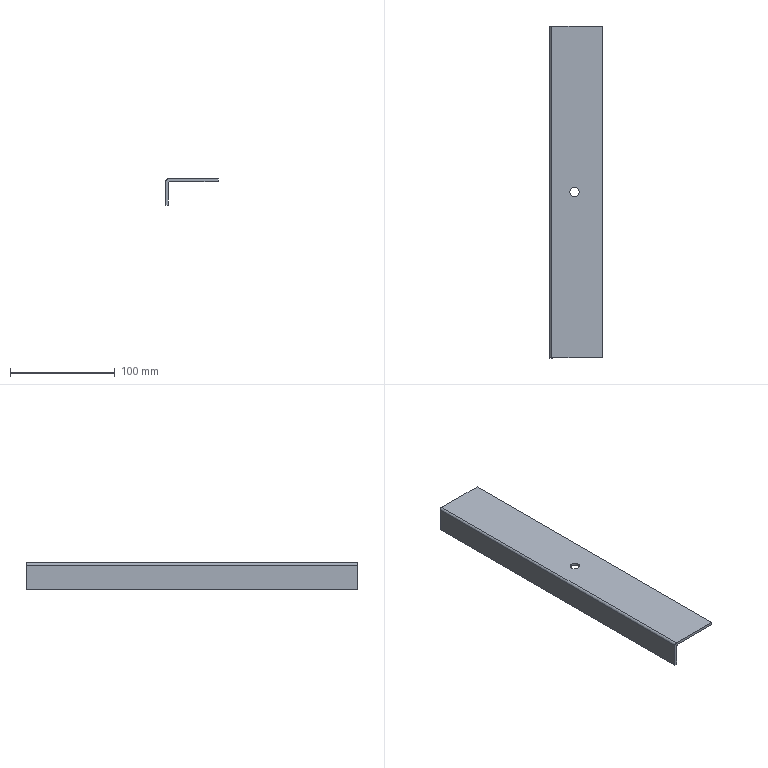Component | SolidWorks | FrameAssembly-1_FrameWeldment-1_SupportPlate-2 | 1 solid | 12 faces | box 50 x 317 x 25 mm | volume 57297 mm3 | plane 8 | cylinder 4 | commonest cylinder face diameters 9 x2 4 x2
STEP:
#1=CARTESIAN_POINT('',(-23.533,4.621,-1.339));
#2=VERTEX_POINT('',#1);
#3=CARTESIAN_POINT('',(-23.533,4.267,-1.339));
#4=VERTEX_POINT('',#3);
#5=CARTESIAN_POINT('',(-23.533,4.444,-1.339));
#6=DIRECTION('',(0.,0.,1.));
#7=DIRECTION('',(0.,-1.,0.));
#8=AXIS2_PLACEMENT_3D('',#5,#6,#7);
#9=CIRCLE('',#8,0.1772);
#10=EDGE_CURVE('',#2,#4,#9,.T.);
#11=ORIENTED_EDGE('',*,*,#10,.F.);
#12=CARTESIAN_POINT('',(-23.533,4.621,-1.24));
#13=VERTEX_POINT('',#12);
#14=CARTESIAN_POINT('',(-23.533,4.621,-1.24));
#15=DIRECTION('',(0.,0.,1.));
#16=VECTOR('',#15,39.37);
#17=LINE('',#14,#16);
#18=EDGE_CURVE('',#2,#13,#17,.T.);
#19=ORIENTED_EDGE('',*,*,#18,.T.);
#20=CARTESIAN_POINT('',(-23.533,4.267,-1.24));
#21=VERTEX_POINT('',#20);
#22=CARTESIAN_POINT('',(-23.533,4.444,-1.24));
#23=DIRECTION('',(0.,0.,1.));
#24=DIRECTION('',(0.,-1.,0.));
#25=AXIS2_PLACEMENT_3D('',#22,#23,#24);
#26=CIRCLE('',#25,0.1772);
#27=EDGE_CURVE('',#13,#21,#26,.T.);
#28=ORIENTED_EDGE('',*,*,#27,.T.);
#29=CARTESIAN_POINT('',(-23.533,4.267,-1.24));
#30=DIRECTION('',(0.,0.,1.));
#31=VECTOR('',#30,39.37);
#32=LINE('',#29,#31);
#33=EDGE_CURVE('',#4,#21,#32,.T.);
#34=ORIENTED_EDGE('',*,*,#33,.F.);
#35=EDGE_LOOP('',(#11,#19,#28,#34));
#36=FACE_OUTER_BOUND('',#35,.T.);
#37=CARTESIAN_POINT('',(-23.533,4.444,-1.24));
#38=DIRECTION('',(0.,0.,1.));
#39=DIRECTION('',(0.,-1.,0.));
#40=AXIS2_PLACEMENT_3D('',#37,#38,#39);
#41=CYLINDRICAL_SURFACE('',#40,0.1772);
#42=ADVANCED_FACE('',(#36),#41,.F.);
#43=CARTESIAN_POINT('',(-24.459,-1.796,-1.319));
#44=VERTEX_POINT('',#43);
#45=CARTESIAN_POINT('',(-24.459,-1.796,-2.224));
#46=VERTEX_POINT('',#45);
#47=CARTESIAN_POINT('',(-24.459,-1.796,-1.319));
#48=DIRECTION('',(-0.,-0.,-1.));
#49=VECTOR('',#48,39.37);
#50=LINE('',#47,#49);
#51=EDGE_CURVE('',#44,#46,#50,.T.);
#52=ORIENTED_EDGE('',*,*,#51,.F.);
#53=CARTESIAN_POINT('',(-24.459,10.684,-1.319));
#54=VERTEX_POINT('',#53);
#55=CARTESIAN_POINT('',(-24.459,10.684,-1.319));
#56=DIRECTION('',(0.,-1.,0.));
#57=VECTOR('',#56,39.37);
#58=LINE('',#55,#57);
#59=EDGE_CURVE('',#54,#44,#58,.T.);
#60=ORIENTED_EDGE('',*,*,#59,.F.);
#61=CARTESIAN_POINT('',(-24.459,10.684,-2.224));
#62=VERTEX_POINT('',#61);
#63=CARTESIAN_POINT('',(-24.459,10.684,-1.319));
#64=DIRECTION('',(-0.,-0.,-1.));
#65=VECTOR('',#64,39.37);
#66=LINE('',#63,#65);
#67=EDGE_CURVE('',#54,#62,#66,.T.);
#68=ORIENTED_EDGE('',*,*,#67,.T.);
#69=CARTESIAN_POINT('',(-24.459,10.684,-2.224));
#70=DIRECTION('',(0.,-1.,0.));
#71=VECTOR('',#70,39.37);
#72=LINE('',#69,#71);
#73=EDGE_CURVE('',#62,#46,#72,.T.);
#74=ORIENTED_EDGE('',*,*,#73,.T.);
#75=EDGE_LOOP('',(#52,#60,#68,#74));
#76=FACE_OUTER_BOUND('',#75,.T.);
#77=CARTESIAN_POINT('',(-24.459,10.684,-1.319));
#78=DIRECTION('',(-1.,-0.,0.));
#79=DIRECTION('',(0.,0.,1.));
#80=AXIS2_PLACEMENT_3D('',#77,#78,#79);
#81=PLANE('',#80);
#82=ADVANCED_FACE('',(#76),#81,.T.);
#83=CARTESIAN_POINT('',(-24.38,-1.796,-1.24));
#84=VERTEX_POINT('',#83);
#85=CARTESIAN_POINT('',(-24.38,-1.796,-1.319));
#86=DIRECTION('',(0.,-1.,0.));
#87=DIRECTION('',(0.,0.,-1.));
#88=AXIS2_PLACEMENT_3D('',#85,#86,#87);
#89=CIRCLE('',#88,0.07874);
#90=EDGE_CURVE('',#84,#44,#89,.T.);
#91=ORIENTED_EDGE('',*,*,#90,.F.);
#92=CARTESIAN_POINT('',(-24.38,10.684,-1.24));
#93=VERTEX_POINT('',#92);
#94=CARTESIAN_POINT('',(-24.38,10.684,-1.24));
#95=DIRECTION('',(0.,-1.,0.));
#96=VECTOR('',#95,39.37);
#97=LINE('',#94,#96);
#98=EDGE_CURVE('',#93,#84,#97,.T.);
#99=ORIENTED_EDGE('',*,*,#98,.F.);
#100=CARTESIAN_POINT('',(-24.38,10.684,-1.319));
#101=DIRECTION('',(0.,-1.,0.));
#102=DIRECTION('',(0.,0.,-1.));
#103=AXIS2_PLACEMENT_3D('',#100,#101,#102);
#104=CIRCLE('',#103,0.07874);
#105=EDGE_CURVE('',#93,#54,#104,.T.);
#106=ORIENTED_EDGE('',*,*,#105,.T.);
#107=ORIENTED_EDGE('',*,*,#59,.T.);
#108=EDGE_LOOP('',(#91,#99,#106,#107));
#109=FACE_OUTER_BOUND('',#108,.T.);
#110=CARTESIAN_POINT('',(-24.38,10.684,-1.319));
#111=DIRECTION('',(0.,-1.,0.));
#112=DIRECTION('',(0.,0.,-1.));
#113=AXIS2_PLACEMENT_3D('',#110,#111,#112);
#114=CYLINDRICAL_SURFACE('',#113,0.07874);
#115=ADVANCED_FACE('',(#109),#114,.T.);
#116=CARTESIAN_POINT('',(-23.533,4.444,-1.24));
#117=DIRECTION('',(0.,0.,1.));
#118=DIRECTION('',(0.,-1.,0.));
#119=AXIS2_PLACEMENT_3D('',#116,#117,#118);
#120=CIRCLE('',#119,0.1772);
#121=EDGE_CURVE('',#21,#13,#120,.T.);
#122=ORIENTED_EDGE('',*,*,#121,.F.);
#123=ORIENTED_EDGE('',*,*,#27,.F.);
#124=EDGE_LOOP('',(#122,#123));
#125=FACE_BOUND('',#124,.T.);
#126=CARTESIAN_POINT('',(-22.49,-1.796,-1.24));
#127=VERTEX_POINT('',#126);
#128=CARTESIAN_POINT('',(-22.49,-1.796,-1.24));
#129=DIRECTION('',(-1.,-0.,0.));
#130=VECTOR('',#129,39.37);
#131=LINE('',#128,#130);
#132=EDGE_CURVE('',#127,#84,#131,.T.);
#133=ORIENTED_EDGE('',*,*,#132,.F.);
#134=CARTESIAN_POINT('',(-22.49,10.684,-1.24));
#135=VERTEX_POINT('',#134);
#136=CARTESIAN_POINT('',(-22.49,10.684,-1.24));
#137=DIRECTION('',(0.,-1.,0.));
#138=VECTOR('',#137,39.37);
#139=LINE('',#136,#138);
#140=EDGE_CURVE('',#135,#127,#139,.T.);
#141=ORIENTED_EDGE('',*,*,#140,.F.);
#142=CARTESIAN_POINT('',(-22.49,10.684,-1.24));
#143=DIRECTION('',(-1.,-0.,0.));
#144=VECTOR('',#143,39.37);
#145=LINE('',#142,#144);
#146=EDGE_CURVE('',#135,#93,#145,.T.);
#147=ORIENTED_EDGE('',*,*,#146,.T.);
#148=ORIENTED_EDGE('',*,*,#98,.T.);
#149=EDGE_LOOP('',(#133,#141,#147,#148));
#150=FACE_OUTER_BOUND('',#149,.T.);
#151=CARTESIAN_POINT('',(-22.49,10.684,-1.24));
#152=DIRECTION('',(0.,0.,1.));
#153=DIRECTION('',(1.,0.,-0.));
#154=AXIS2_PLACEMENT_3D('',#151,#152,#153);
#155=PLANE('',#154);
#156=ADVANCED_FACE('',(#125,#150),#155,.T.);
#157=CARTESIAN_POINT('',(-22.49,-1.796,-1.339));
#158=VERTEX_POINT('',#157);
#159=CARTESIAN_POINT('',(-22.49,10.684,-1.339));
#160=VERTEX_POINT('',#159);
#161=CARTESIAN_POINT('',(-22.49,-1.796,-1.339));
#162=DIRECTION('',(-0.,1.,-0.));
#163=VECTOR('',#162,39.37);
#164=LINE('',#161,#163);
#165=EDGE_CURVE('',#158,#160,#164,.T.);
#166=ORIENTED_EDGE('',*,*,#165,.T.);
#167=CARTESIAN_POINT('',(-22.49,10.684,-2.224));
#168=DIRECTION('',(0.,0.,1.));
#169=VECTOR('',#168,39.37);
#170=LINE('',#167,#169);
#171=EDGE_CURVE('',#160,#135,#170,.T.);
#172=ORIENTED_EDGE('',*,*,#171,.T.);
#173=ORIENTED_EDGE('',*,*,#140,.T.);
#174=CARTESIAN_POINT('',(-22.49,-1.796,-2.224));
#175=DIRECTION('',(0.,0.,1.));
#176=VECTOR('',#175,39.37);
#177=LINE('',#174,#176);
#178=EDGE_CURVE('',#158,#127,#177,.T.);
#179=ORIENTED_EDGE('',*,*,#178,.F.);
#180=EDGE_LOOP('',(#166,#172,#173,#179));
#181=FACE_OUTER_BOUND('',#180,.T.);
#182=CARTESIAN_POINT('',(-22.49,10.684,-2.224));
#183=DIRECTION('',(1.,0.,-0.));
#184=DIRECTION('',(-0.,1.,-0.));
#185=AXIS2_PLACEMENT_3D('',#182,#183,#184);
#186=PLANE('',#185);
#187=ADVANCED_FACE('',(#181),#186,.T.);
#188=CARTESIAN_POINT('',(-24.36,-1.796,-2.224));
#189=VERTEX_POINT('',#188);
#190=CARTESIAN_POINT('',(-24.36,10.684,-2.224));
#191=VERTEX_POINT('',#190);
#192=CARTESIAN_POINT('',(-24.36,-1.796,-2.224));
#193=DIRECTION('',(-0.,1.,-0.));
#194=VECTOR('',#193,39.37);
#195=LINE('',#192,#194);
#196=EDGE_CURVE('',#189,#191,#195,.T.);
#197=ORIENTED_EDGE('',*,*,#196,.F.);
#198=CARTESIAN_POINT('',(-24.459,-1.796,-2.224));
#199=DIRECTION('',(1.,0.,-0.));
#200=VECTOR('',#199,39.37);
#201=LINE('',#198,#200);
#202=EDGE_CURVE('',#46,#189,#201,.T.);
#203=ORIENTED_EDGE('',*,*,#202,.F.);
#204=ORIENTED_EDGE('',*,*,#73,.F.);
#205=CARTESIAN_POINT('',(-24.459,10.684,-2.224));
#206=DIRECTION('',(1.,0.,-0.));
#207=VECTOR('',#206,39.37);
#208=LINE('',#205,#207);
#209=EDGE_CURVE('',#62,#191,#208,.T.);
#210=ORIENTED_EDGE('',*,*,#209,.T.);
#211=EDGE_LOOP('',(#197,#203,#204,#210));
#212=FACE_OUTER_BOUND('',#211,.T.);
#213=CARTESIAN_POINT('',(-24.459,10.684,-2.224));
#214=DIRECTION('',(-0.,-0.,-1.));
#215=DIRECTION('',(-0.,1.,-0.));
#216=AXIS2_PLACEMENT_3D('',#213,#214,#215);
#217=PLANE('',#216);
#218=ADVANCED_FACE('',(#212),#217,.T.);
#219=ORIENTED_EDGE('',*,*,#171,.F.);
#220=CARTESIAN_POINT('',(-24.281,10.684,-1.339));
#221=VERTEX_POINT('',#220);
#222=CARTESIAN_POINT('',(-24.281,10.684,-1.339));
#223=DIRECTION('',(1.,0.,-0.));
#224=VECTOR('',#223,39.37);
#225=LINE('',#222,#224);
#226=EDGE_CURVE('',#221,#160,#225,.T.);
#227=ORIENTED_EDGE('',*,*,#226,.F.);
#228=CARTESIAN_POINT('',(-24.36,10.684,-1.417));
#229=VERTEX_POINT('',#228);
#230=CARTESIAN_POINT('',(-24.281,10.684,-1.417));
#231=DIRECTION('',(-0.,1.,-0.));
#232=DIRECTION('',(0.,0.,1.));
#233=AXIS2_PLACEMENT_3D('',#230,#231,#232);
#234=CIRCLE('',#233,0.07874);
#235=EDGE_CURVE('',#229,#221,#234,.T.);
#236=ORIENTED_EDGE('',*,*,#235,.F.);
#237=CARTESIAN_POINT('',(-24.36,10.684,-2.224));
#238=DIRECTION('',(0.,0.,1.));
#239=VECTOR('',#238,39.37);
#240=LINE('',#237,#239);
#241=EDGE_CURVE('',#191,#229,#240,.T.);
#242=ORIENTED_EDGE('',*,*,#241,.F.);
#243=ORIENTED_EDGE('',*,*,#209,.F.);
#244=ORIENTED_EDGE('',*,*,#67,.F.);
#245=ORIENTED_EDGE('',*,*,#105,.F.);
#246=ORIENTED_EDGE('',*,*,#146,.F.);
#247=EDGE_LOOP('',(#219,#227,#236,#242,#243,#244,#245,#246));
#248=FACE_OUTER_BOUND('',#247,.T.);
#249=CARTESIAN_POINT('',(-24.38,10.684,-1.319));
#250=DIRECTION('',(0.,-1.,0.));
#251=DIRECTION('',(-0.,-0.,-1.));
#252=AXIS2_PLACEMENT_3D('',#249,#250,#251);
#253=PLANE('',#252);
#254=ADVANCED_FACE('',(#248),#253,.F.);
#255=CARTESIAN_POINT('',(-24.281,-1.796,-1.339));
#256=VERTEX_POINT('',#255);
#257=CARTESIAN_POINT('',(-24.281,-1.796,-1.339));
#258=DIRECTION('',(1.,0.,-0.));
#259=VECTOR('',#258,39.37);
#260=LINE('',#257,#259);
#261=EDGE_CURVE('',#256,#158,#260,.T.);
#262=ORIENTED_EDGE('',*,*,#261,.T.);
#263=ORIENTED_EDGE('',*,*,#178,.T.);
#264=ORIENTED_EDGE('',*,*,#132,.T.);
#265=ORIENTED_EDGE('',*,*,#90,.T.);
#266=ORIENTED_EDGE('',*,*,#51,.T.);
#267=ORIENTED_EDGE('',*,*,#202,.T.);
#268=CARTESIAN_POINT('',(-24.36,-1.796,-1.417));
#269=VERTEX_POINT('',#268);
#270=CARTESIAN_POINT('',(-24.36,-1.796,-2.224));
#271=DIRECTION('',(0.,0.,1.));
#272=VECTOR('',#271,39.37);
#273=LINE('',#270,#272);
#274=EDGE_CURVE('',#189,#269,#273,.T.);
#275=ORIENTED_EDGE('',*,*,#274,.T.);
#276=CARTESIAN_POINT('',(-24.281,-1.796,-1.417));
#277=DIRECTION('',(-0.,1.,-0.));
#278=DIRECTION('',(0.,0.,1.));
#279=AXIS2_PLACEMENT_3D('',#276,#277,#278);
#280=CIRCLE('',#279,0.07874);
#281=EDGE_CURVE('',#269,#256,#280,.T.);
#282=ORIENTED_EDGE('',*,*,#281,.T.);
#283=EDGE_LOOP('',(#262,#263,#264,#265,#266,#267,#275,#282));
#284=FACE_OUTER_BOUND('',#283,.T.);
#285=CARTESIAN_POINT('',(-24.38,-1.796,-1.319));
#286=DIRECTION('',(0.,-1.,0.));
#287=DIRECTION('',(-0.,-0.,-1.));
#288=AXIS2_PLACEMENT_3D('',#285,#286,#287);
#289=PLANE('',#288);
#290=ADVANCED_FACE('',(#284),#289,.T.);
#291=CARTESIAN_POINT('',(-23.533,4.444,-1.339));
#292=DIRECTION('',(0.,0.,1.));
#293=DIRECTION('',(0.,-1.,0.));
#294=AXIS2_PLACEMENT_3D('',#291,#292,#293);
#295=CIRCLE('',#294,0.1772);
#296=EDGE_CURVE('',#4,#2,#295,.T.);
#297=ORIENTED_EDGE('',*,*,#296,.T.);
#298=ORIENTED_EDGE('',*,*,#10,.T.);
#299=EDGE_LOOP('',(#297,#298));
#300=FACE_BOUND('',#299,.T.);
#301=ORIENTED_EDGE('',*,*,#226,.T.);
#302=ORIENTED_EDGE('',*,*,#165,.F.);
#303=ORIENTED_EDGE('',*,*,#261,.F.);
#304=CARTESIAN_POINT('',(-24.281,-1.796,-1.339));
#305=DIRECTION('',(-0.,1.,-0.));
#306=VECTOR('',#305,39.37);
#307=LINE('',#304,#306);
#308=EDGE_CURVE('',#256,#221,#307,.T.);
#309=ORIENTED_EDGE('',*,*,#308,.T.);
#310=EDGE_LOOP('',(#301,#302,#303,#309));
#311=FACE_OUTER_BOUND('',#310,.T.);
#312=CARTESIAN_POINT('',(-24.281,-1.796,-1.339));
#313=DIRECTION('',(0.,0.,1.));
#314=DIRECTION('',(0.,-1.,0.));
#315=AXIS2_PLACEMENT_3D('',#312,#313,#314);
#316=PLANE('',#315);
#317=ADVANCED_FACE('',(#300,#311),#316,.F.);
#318=ORIENTED_EDGE('',*,*,#235,.T.);
#319=ORIENTED_EDGE('',*,*,#308,.F.);
#320=ORIENTED_EDGE('',*,*,#281,.F.);
#321=CARTESIAN_POINT('',(-24.36,-1.796,-1.417));
#322=DIRECTION('',(-0.,1.,-0.));
#323=VECTOR('',#322,39.37);
#324=LINE('',#321,#323);
#325=EDGE_CURVE('',#269,#229,#324,.T.);
#326=ORIENTED_EDGE('',*,*,#325,.T.);
#327=EDGE_LOOP('',(#318,#319,#320,#326));
#328=FACE_OUTER_BOUND('',#327,.T.);
#329=CARTESIAN_POINT('',(-24.281,-1.796,-1.417));
#330=DIRECTION('',(-0.,1.,-0.));
#331=DIRECTION('',(0.,0.,1.));
#332=AXIS2_PLACEMENT_3D('',#329,#330,#331);
#333=CYLINDRICAL_SURFACE('',#332,0.07874);
#334=ADVANCED_FACE('',(#328),#333,.F.);
#335=ORIENTED_EDGE('',*,*,#241,.T.);
#336=ORIENTED_EDGE('',*,*,#325,.F.);
#337=ORIENTED_EDGE('',*,*,#274,.F.);
#338=ORIENTED_EDGE('',*,*,#196,.T.);
#339=EDGE_LOOP('',(#335,#336,#337,#338));
#340=FACE_OUTER_BOUND('',#339,.T.);
#341=CARTESIAN_POINT('',(-24.36,-1.796,-2.224));
#342=DIRECTION('',(-1.,-0.,0.));
#343=DIRECTION('',(0.,0.,1.));
#344=AXIS2_PLACEMENT_3D('',#341,#342,#343);
#345=PLANE('',#344);
#346=ADVANCED_FACE('',(#340),#345,.F.);
#347=ORIENTED_EDGE('',*,*,#18,.F.);
#348=ORIENTED_EDGE('',*,*,#296,.F.);
#349=ORIENTED_EDGE('',*,*,#33,.T.);
#350=ORIENTED_EDGE('',*,*,#121,.T.);
#351=EDGE_LOOP('',(#347,#348,#349,#350));
#352=FACE_OUTER_BOUND('',#351,.T.);
#353=CARTESIAN_POINT('',(-23.533,4.444,-1.24));
#354=DIRECTION('',(0.,0.,1.));
#355=DIRECTION('',(0.,-1.,0.));
#356=AXIS2_PLACEMENT_3D('',#353,#354,#355);
#357=CYLINDRICAL_SURFACE('',#356,0.1772);
#358=ADVANCED_FACE('',(#352),#357,.F.);
#359=CLOSED_SHELL('',(#42,#82,#115,#156,#187,#218,#254,#290,#317,#334,#346,#358));
#360=MANIFOLD_SOLID_BREP('',#359);
#361=CARTESIAN_POINT('',(0.,0.,0.));
#362=DIRECTION('',(0.,0.,1.));
#363=DIRECTION('',(1.,0.,0.));
#364=AXIS2_PLACEMENT_3D('',#361,#362,#363);
#365=(LENGTH_UNIT()NAMED_UNIT(*)SI_UNIT($,.METRE.));
#366=LENGTH_MEASURE_WITH_UNIT(LENGTH_MEASURE(0.0254),#365);
#367=DIMENSIONAL_EXPONENTS(1.,0.,0.,0.,0.,0.,0.);
#368=(CONVERSION_BASED_UNIT('',#366)LENGTH_UNIT()NAMED_UNIT(#367));
#369=UNCERTAINTY_MEASURE_WITH_UNIT(LENGTH_MEASURE(0.00001),#368,'','');
#370=(NAMED_UNIT(*)PLANE_ANGLE_UNIT()SI_UNIT($,.RADIAN.));
#371=(NAMED_UNIT(*)SI_UNIT($,.STERADIAN.)SOLID_ANGLE_UNIT());
#372=(GEOMETRIC_REPRESENTATION_CONTEXT(3)GLOBAL_UNCERTAINTY_ASSIGNED_CONTEXT((#369))GLOBAL_UNIT_ASSIGNED_CONTEXT((#368,#370,#371))REPRESENTATION_CONTEXT('',''));
#373=ADVANCED_BREP_SHAPE_REPRESENTATION('',(#360,#364),#372);
#374=COLOUR_RGB('',0.7922,0.8196,0.9333);
#375=FILL_AREA_STYLE_COLOUR('',#374);
#376=FILL_AREA_STYLE('',(#375));
#377=SURFACE_STYLE_FILL_AREA(#376);
#378=SURFACE_SIDE_STYLE('',(#377));
#379=SURFACE_STYLE_USAGE(.BOTH.,#378);
#380=PRESENTATION_STYLE_ASSIGNMENT((#379));
#381=STYLED_ITEM('',(#380),#360);
#382=PRESENTATION_LAYER_ASSIGNMENT('','',(#381));
#383=(LENGTH_UNIT()NAMED_UNIT(*)SI_UNIT($,.METRE.));
#384=LENGTH_MEASURE_WITH_UNIT(LENGTH_MEASURE(0.0254),#383);
#385=DIMENSIONAL_EXPONENTS(1.,0.,0.,0.,0.,0.,0.);
#386=(CONVERSION_BASED_UNIT('',#384)LENGTH_UNIT()NAMED_UNIT(#385));
#387=UNCERTAINTY_MEASURE_WITH_UNIT(LENGTH_MEASURE(0.00001),#386,'','');
#388=(NAMED_UNIT(*)PLANE_ANGLE_UNIT()SI_UNIT($,.RADIAN.));
#389=(NAMED_UNIT(*)SI_UNIT($,.STERADIAN.)SOLID_ANGLE_UNIT());
#390=(GEOMETRIC_REPRESENTATION_CONTEXT(3)GLOBAL_UNCERTAINTY_ASSIGNED_CONTEXT((#387))GLOBAL_UNIT_ASSIGNED_CONTEXT((#386,#388,#389))REPRESENTATION_CONTEXT('',''));
#391=MECHANICAL_DESIGN_GEOMETRIC_PRESENTATION_REPRESENTATION('',(#381),#390);